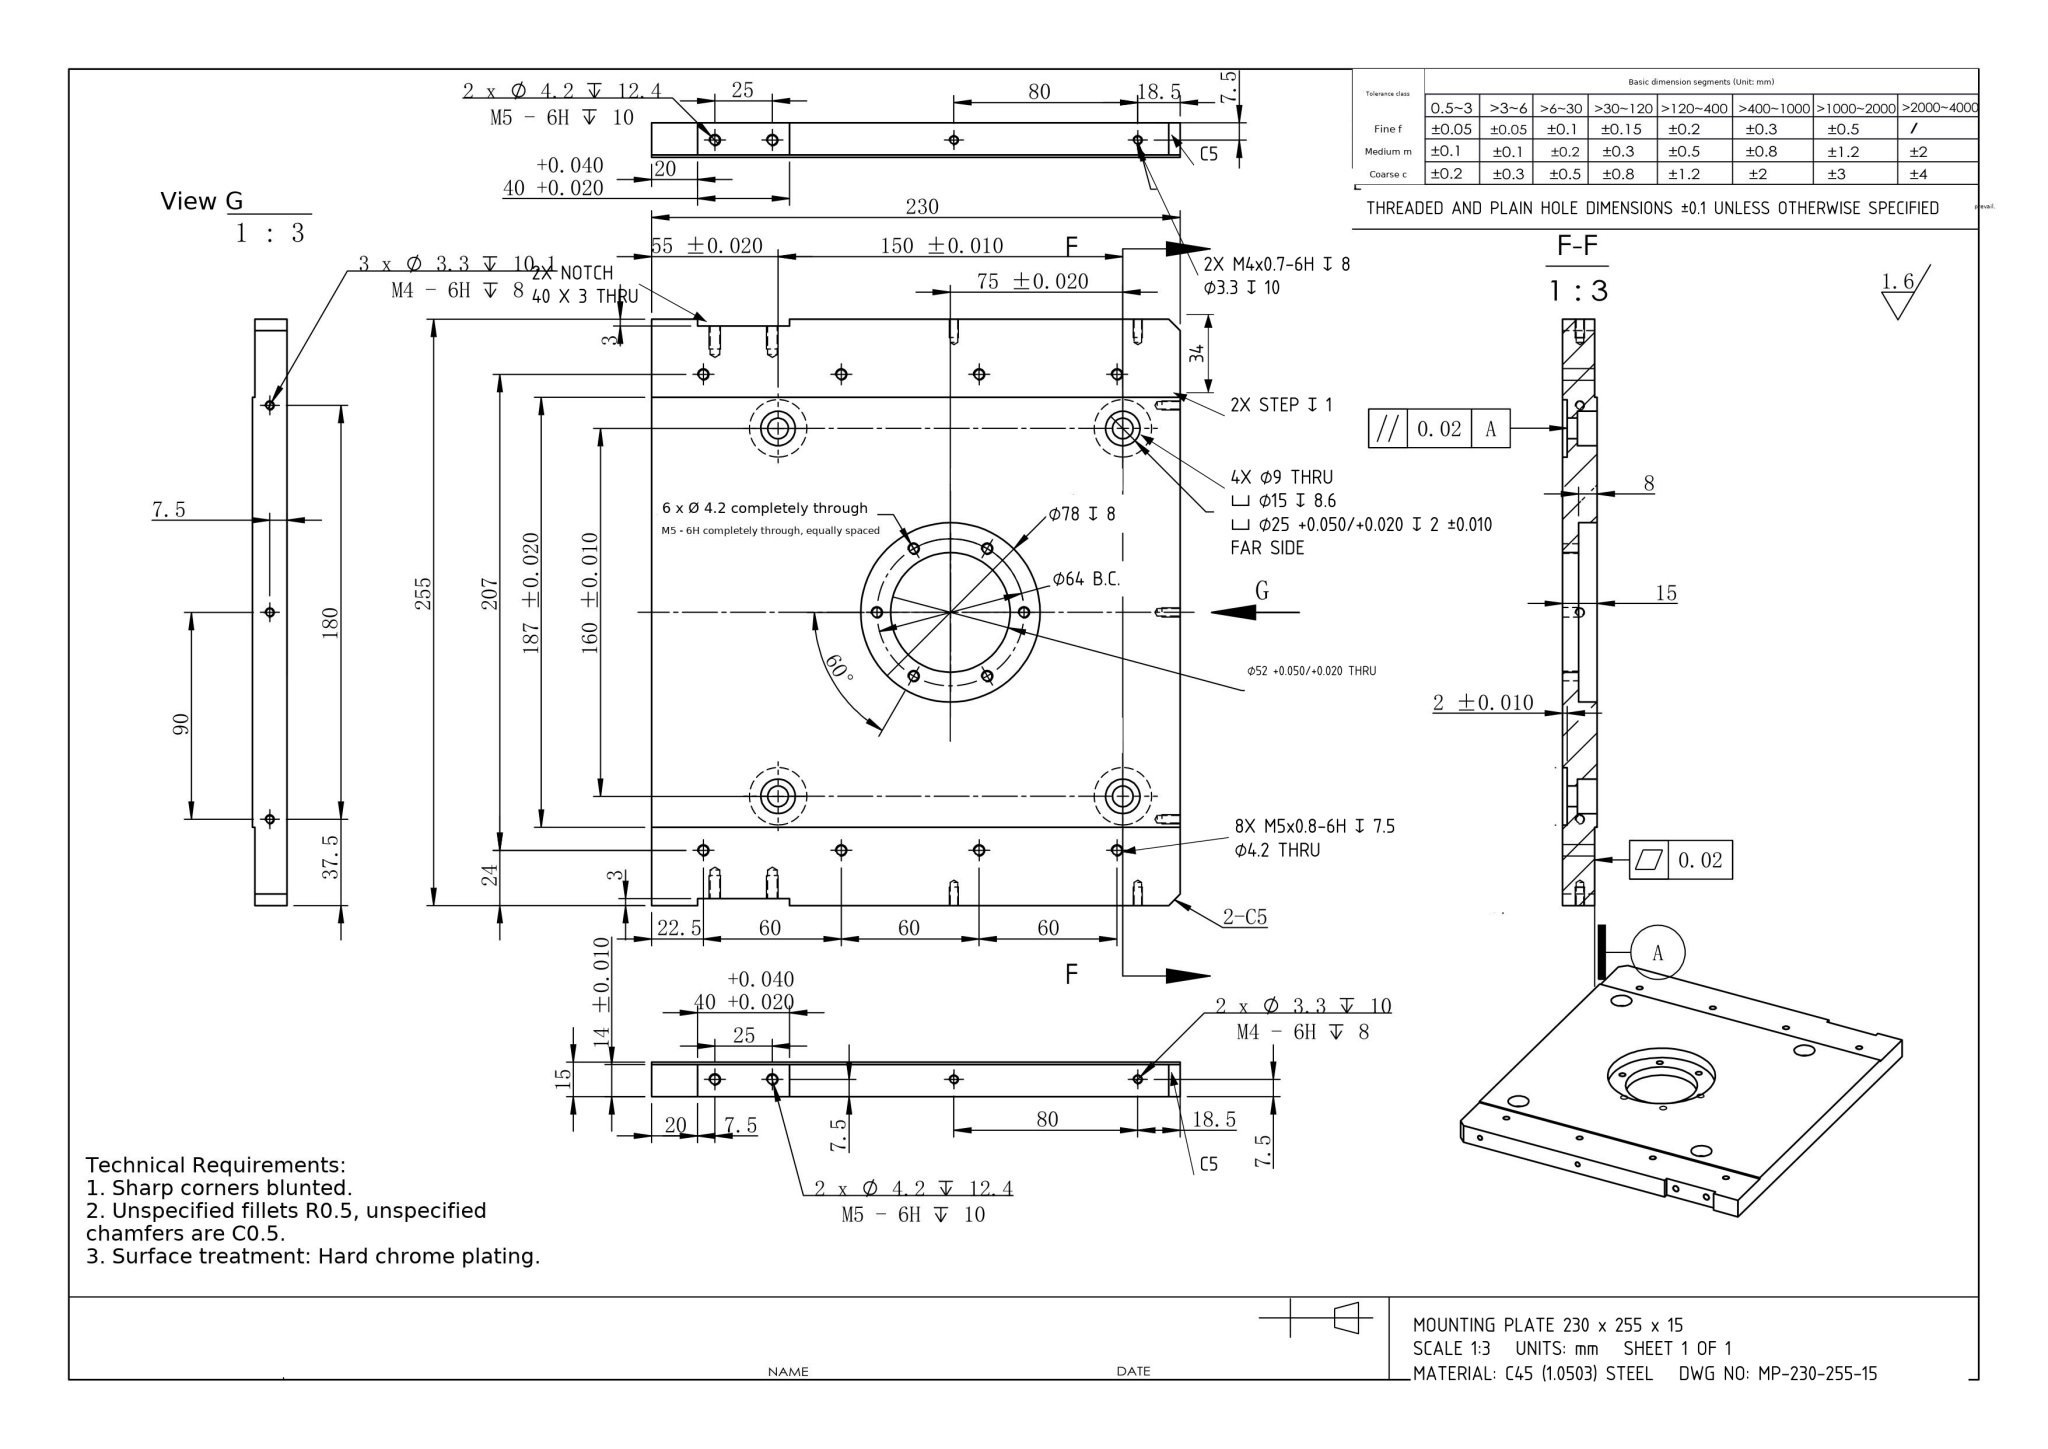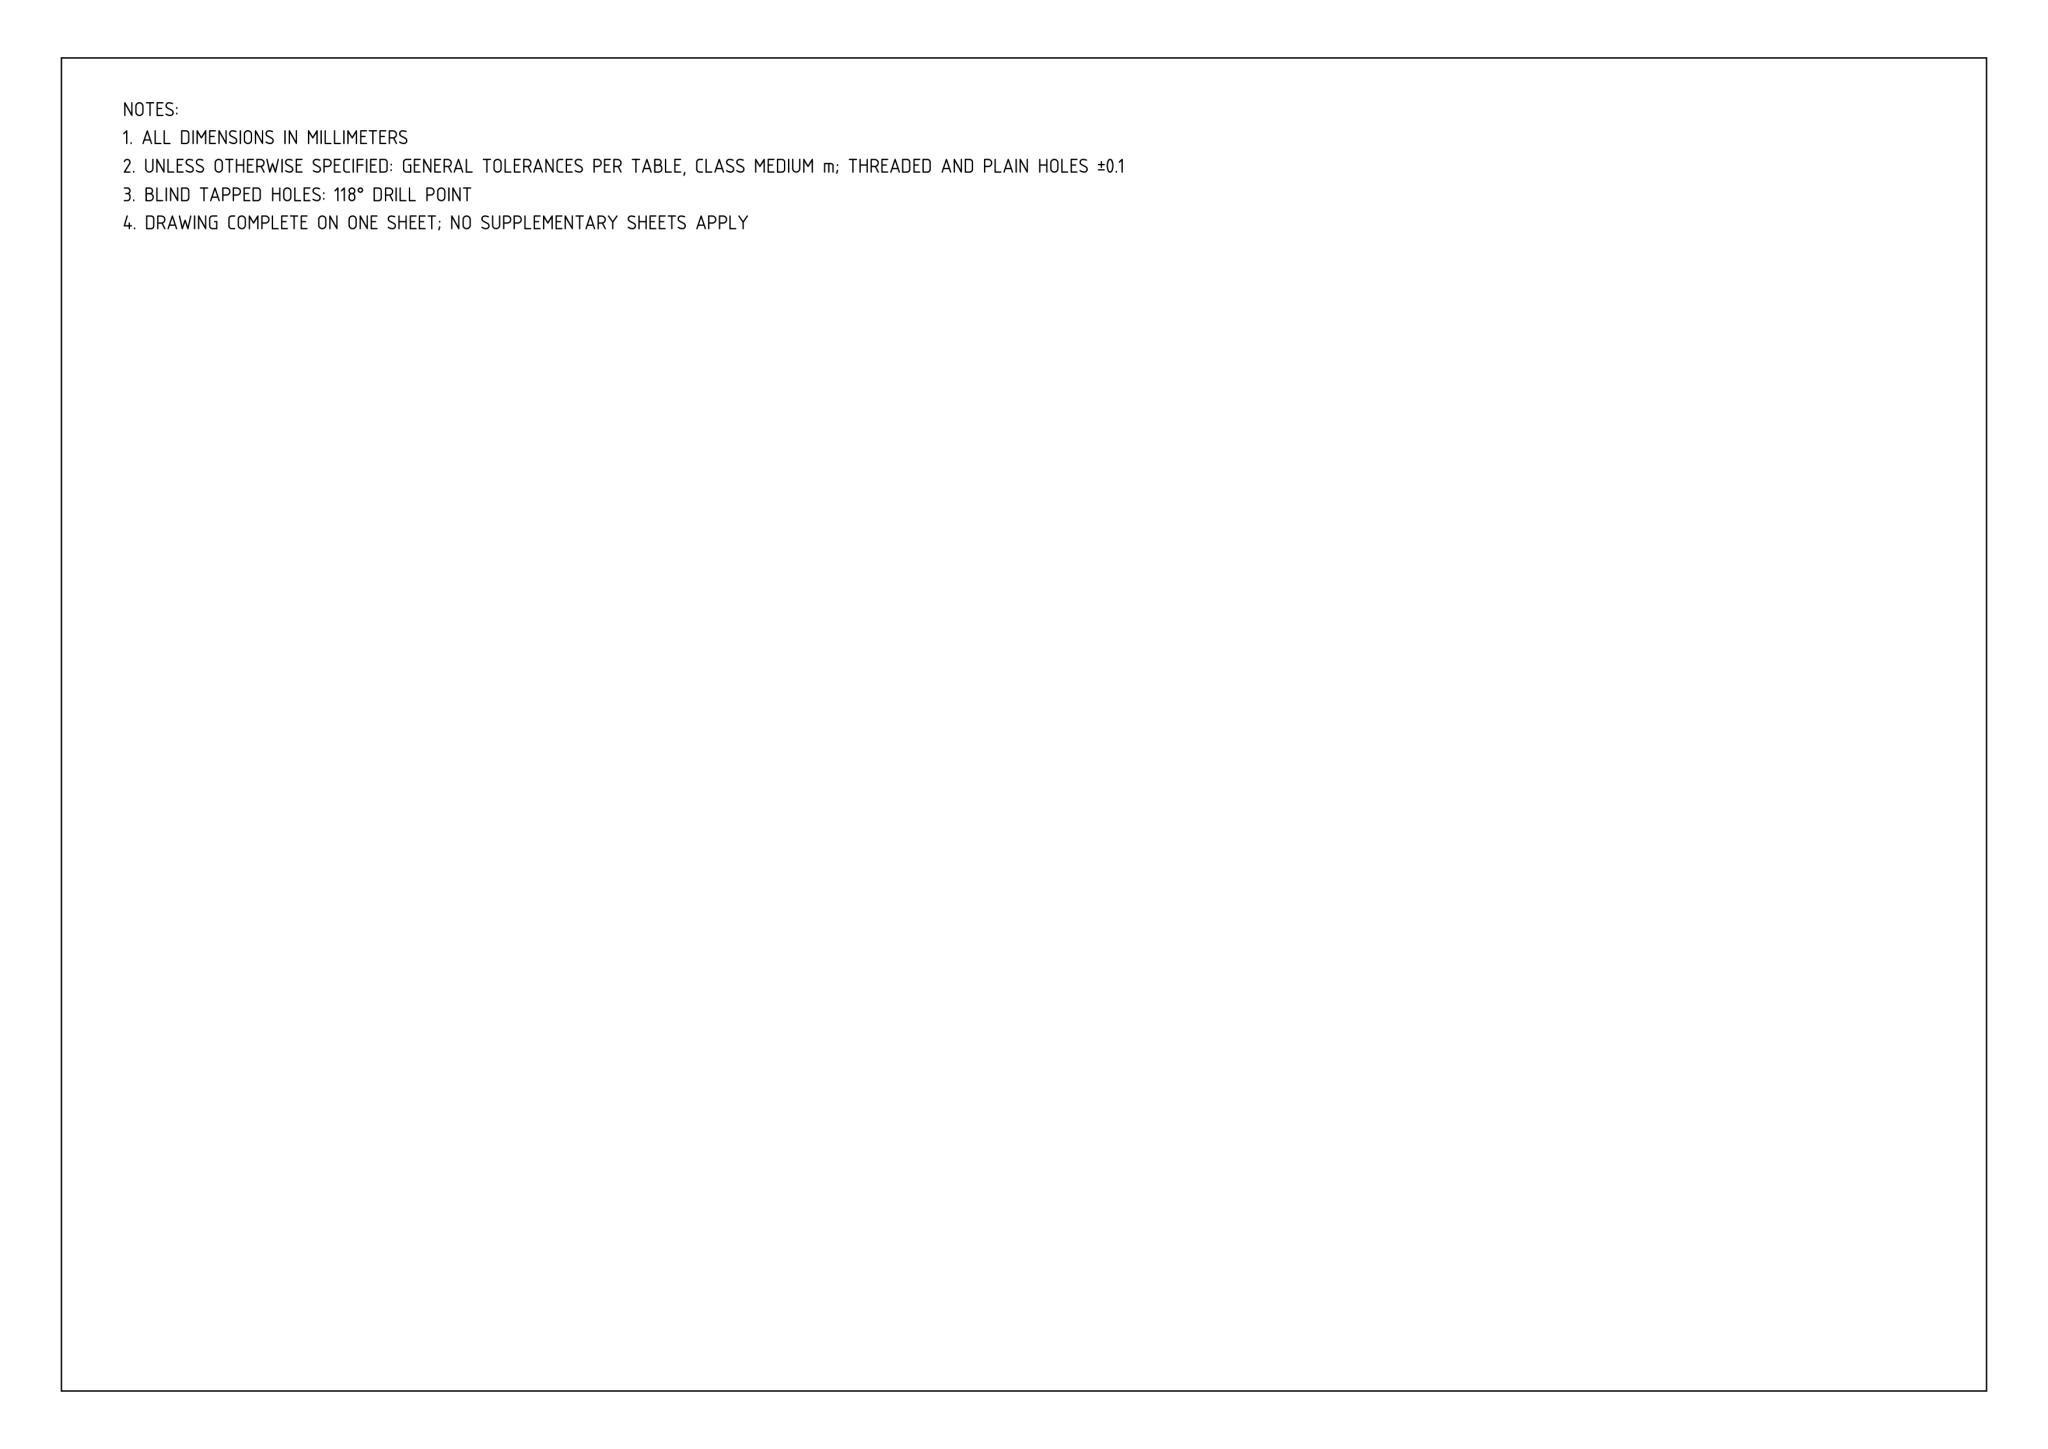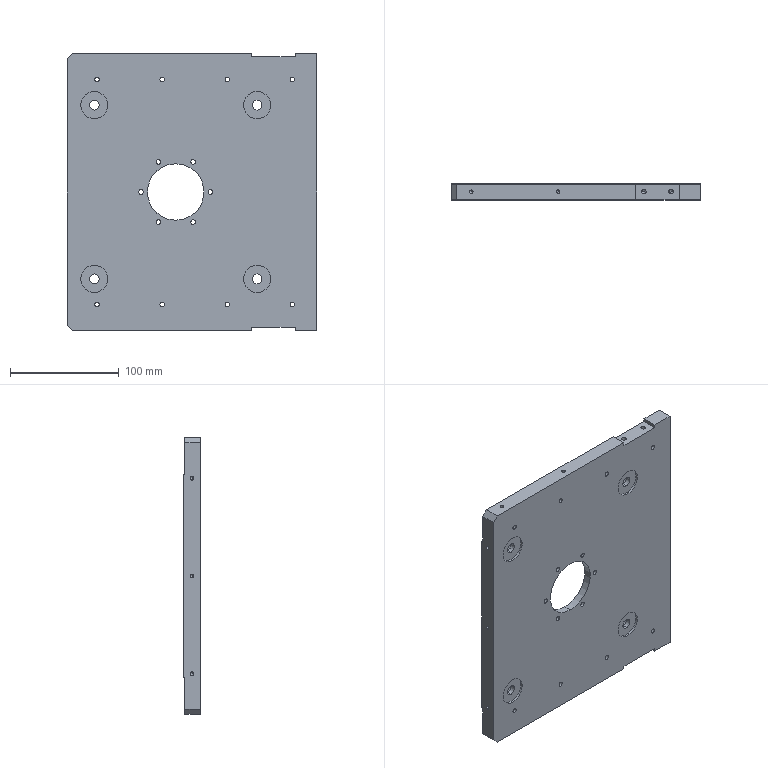Part | NX | mm | 1 solid | 129 faces | box 230 x 15 x 255 mm | volume 792715 mm3 | cylinder 78 | plane 29 | cone 22 | commonest cylinder face diameters 4.2 x36 3.3 x14 15 x8 9 x8 25 x8 52 x2 78 x2